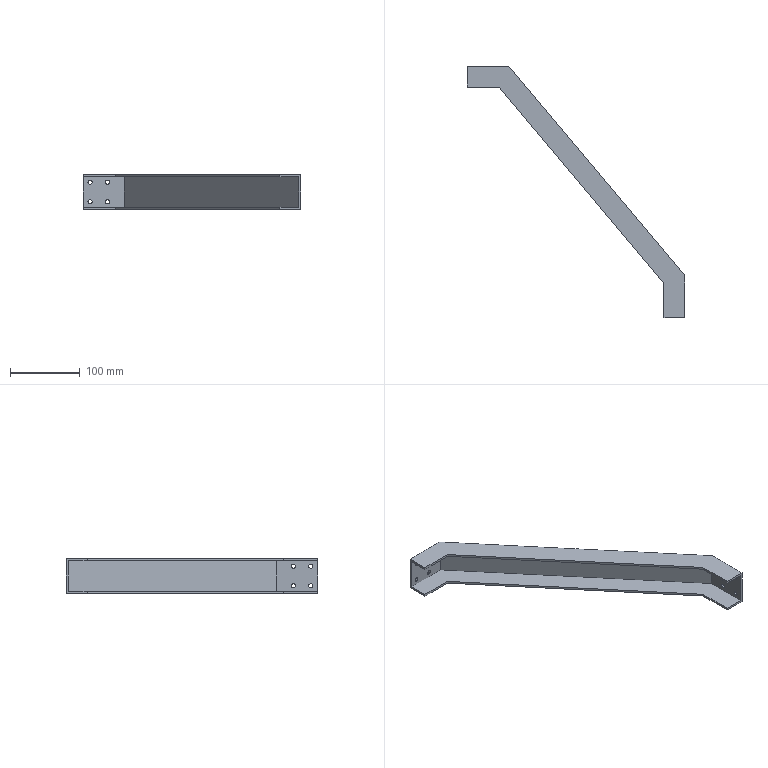Component | SolidWorks | BaffleFixingBracket-1 | 1 solid | 34 faces | box 311.73 x 360 x 50 mm | volume 154135 mm3 | plane 18 | cylinder 16 | commonest cylinder face diameters 6 x16
STEP:
#1=COLOUR_RGB('',0.7922,0.8196,0.9333);
#2=FILL_AREA_STYLE_COLOUR('',#1);
#3=FILL_AREA_STYLE('',(#2));
#4=SURFACE_STYLE_FILL_AREA(#3);
#5=SURFACE_SIDE_STYLE('',(#4));
#6=SURFACE_STYLE_USAGE(.BOTH.,#5);
#7=PRESENTATION_STYLE_ASSIGNMENT((#6));
#8=CARTESIAN_POINT('',(-24.578,20.455,-13.277));
#9=VERTEX_POINT('',#8);
#10=CARTESIAN_POINT('',(-24.342,20.455,-13.277));
#11=VERTEX_POINT('',#10);
#12=CARTESIAN_POINT('',(-24.46,20.455,-13.277));
#13=DIRECTION('',(0.,-1.,0.));
#14=DIRECTION('',(1.,0.,0.));
#15=AXIS2_PLACEMENT_3D('',#12,#13,#14);
#16=CIRCLE('',#15,0.1181);
#17=EDGE_CURVE('',#9,#11,#16,.T.);
#18=ORIENTED_EDGE('',*,*,#17,.F.);
#19=CARTESIAN_POINT('',(-24.578,20.337,-13.277));
#20=VERTEX_POINT('',#19);
#21=CARTESIAN_POINT('',(-24.578,20.455,-13.277));
#22=DIRECTION('',(0.,-1.,0.));
#23=VECTOR('',#22,39.37);
#24=LINE('',#21,#23);
#25=EDGE_CURVE('',#9,#20,#24,.T.);
#26=ORIENTED_EDGE('',*,*,#25,.T.);
#27=CARTESIAN_POINT('',(-24.342,20.337,-13.277));
#28=VERTEX_POINT('',#27);
#29=CARTESIAN_POINT('',(-24.46,20.337,-13.277));
#30=DIRECTION('',(0.,-1.,0.));
#31=DIRECTION('',(1.,0.,0.));
#32=AXIS2_PLACEMENT_3D('',#29,#30,#31);
#33=CIRCLE('',#32,0.1181);
#34=EDGE_CURVE('',#20,#28,#33,.T.);
#35=ORIENTED_EDGE('',*,*,#34,.T.);
#36=CARTESIAN_POINT('',(-24.342,20.455,-13.277));
#37=DIRECTION('',(0.,-1.,0.));
#38=VECTOR('',#37,39.37);
#39=LINE('',#36,#38);
#40=EDGE_CURVE('',#11,#28,#39,.T.);
#41=ORIENTED_EDGE('',*,*,#40,.F.);
#42=EDGE_LOOP('',(#18,#26,#35,#41));
#43=FACE_OUTER_BOUND('',#42,.T.);
#44=CARTESIAN_POINT('',(-24.46,20.455,-13.277));
#45=DIRECTION('',(0.,-1.,0.));
#46=DIRECTION('',(1.,0.,0.));
#47=AXIS2_PLACEMENT_3D('',#44,#45,#46);
#48=CYLINDRICAL_SURFACE('',#47,0.1181);
#49=ADVANCED_FACE('',(#43),#48,.F.);
#50=CARTESIAN_POINT('',(-24.578,20.455,-12.174));
#51=VERTEX_POINT('',#50);
#52=CARTESIAN_POINT('',(-24.342,20.455,-12.174));
#53=VERTEX_POINT('',#52);
#54=CARTESIAN_POINT('',(-24.46,20.455,-12.174));
#55=DIRECTION('',(0.,-1.,0.));
#56=DIRECTION('',(1.,0.,0.));
#57=AXIS2_PLACEMENT_3D('',#54,#55,#56);
#58=CIRCLE('',#57,0.1181);
#59=EDGE_CURVE('',#51,#53,#58,.T.);
#60=ORIENTED_EDGE('',*,*,#59,.F.);
#61=CARTESIAN_POINT('',(-24.578,20.337,-12.174));
#62=VERTEX_POINT('',#61);
#63=CARTESIAN_POINT('',(-24.578,20.455,-12.174));
#64=DIRECTION('',(0.,-1.,0.));
#65=VECTOR('',#64,39.37);
#66=LINE('',#63,#65);
#67=EDGE_CURVE('',#51,#62,#66,.T.);
#68=ORIENTED_EDGE('',*,*,#67,.T.);
#69=CARTESIAN_POINT('',(-24.342,20.337,-12.174));
#70=VERTEX_POINT('',#69);
#71=CARTESIAN_POINT('',(-24.46,20.337,-12.174));
#72=DIRECTION('',(0.,-1.,0.));
#73=DIRECTION('',(1.,0.,0.));
#74=AXIS2_PLACEMENT_3D('',#71,#72,#73);
#75=CIRCLE('',#74,0.1181);
#76=EDGE_CURVE('',#62,#70,#75,.T.);
#77=ORIENTED_EDGE('',*,*,#76,.T.);
#78=CARTESIAN_POINT('',(-24.342,20.455,-12.174));
#79=DIRECTION('',(0.,-1.,0.));
#80=VECTOR('',#79,39.37);
#81=LINE('',#78,#80);
#82=EDGE_CURVE('',#53,#70,#81,.T.);
#83=ORIENTED_EDGE('',*,*,#82,.F.);
#84=EDGE_LOOP('',(#60,#68,#77,#83));
#85=FACE_OUTER_BOUND('',#84,.T.);
#86=CARTESIAN_POINT('',(-24.46,20.455,-12.174));
#87=DIRECTION('',(0.,-1.,0.));
#88=DIRECTION('',(1.,0.,0.));
#89=AXIS2_PLACEMENT_3D('',#86,#87,#88);
#90=CYLINDRICAL_SURFACE('',#89,0.1181);
#91=ADVANCED_FACE('',(#85),#90,.F.);
#92=CARTESIAN_POINT('',(-23.594,20.455,-13.277));
#93=VERTEX_POINT('',#92);
#94=CARTESIAN_POINT('',(-23.357,20.455,-13.277));
#95=VERTEX_POINT('',#94);
#96=CARTESIAN_POINT('',(-23.476,20.455,-13.277));
#97=DIRECTION('',(0.,-1.,0.));
#98=DIRECTION('',(1.,0.,0.));
#99=AXIS2_PLACEMENT_3D('',#96,#97,#98);
#100=CIRCLE('',#99,0.1181);
#101=EDGE_CURVE('',#93,#95,#100,.T.);
#102=ORIENTED_EDGE('',*,*,#101,.F.);
#103=CARTESIAN_POINT('',(-23.594,20.337,-13.277));
#104=VERTEX_POINT('',#103);
#105=CARTESIAN_POINT('',(-23.594,20.455,-13.277));
#106=DIRECTION('',(0.,-1.,0.));
#107=VECTOR('',#106,39.37);
#108=LINE('',#105,#107);
#109=EDGE_CURVE('',#93,#104,#108,.T.);
#110=ORIENTED_EDGE('',*,*,#109,.T.);
#111=CARTESIAN_POINT('',(-23.357,20.337,-13.277));
#112=VERTEX_POINT('',#111);
#113=CARTESIAN_POINT('',(-23.476,20.337,-13.277));
#114=DIRECTION('',(0.,-1.,0.));
#115=DIRECTION('',(1.,0.,0.));
#116=AXIS2_PLACEMENT_3D('',#113,#114,#115);
#117=CIRCLE('',#116,0.1181);
#118=EDGE_CURVE('',#104,#112,#117,.T.);
#119=ORIENTED_EDGE('',*,*,#118,.T.);
#120=CARTESIAN_POINT('',(-23.357,20.455,-13.277));
#121=DIRECTION('',(0.,-1.,0.));
#122=VECTOR('',#121,39.37);
#123=LINE('',#120,#122);
#124=EDGE_CURVE('',#95,#112,#123,.T.);
#125=ORIENTED_EDGE('',*,*,#124,.F.);
#126=EDGE_LOOP('',(#102,#110,#119,#125));
#127=FACE_OUTER_BOUND('',#126,.T.);
#128=CARTESIAN_POINT('',(-23.476,20.455,-13.277));
#129=DIRECTION('',(0.,-1.,0.));
#130=DIRECTION('',(1.,0.,0.));
#131=AXIS2_PLACEMENT_3D('',#128,#129,#130);
#132=CYLINDRICAL_SURFACE('',#131,0.1181);
#133=ADVANCED_FACE('',(#127),#132,.F.);
#134=CARTESIAN_POINT('',(-23.594,20.455,-12.174));
#135=VERTEX_POINT('',#134);
#136=CARTESIAN_POINT('',(-23.357,20.455,-12.174));
#137=VERTEX_POINT('',#136);
#138=CARTESIAN_POINT('',(-23.476,20.455,-12.174));
#139=DIRECTION('',(0.,-1.,0.));
#140=DIRECTION('',(1.,0.,0.));
#141=AXIS2_PLACEMENT_3D('',#138,#139,#140);
#142=CIRCLE('',#141,0.1181);
#143=EDGE_CURVE('',#135,#137,#142,.T.);
#144=ORIENTED_EDGE('',*,*,#143,.F.);
#145=CARTESIAN_POINT('',(-23.594,20.337,-12.174));
#146=VERTEX_POINT('',#145);
#147=CARTESIAN_POINT('',(-23.594,20.455,-12.174));
#148=DIRECTION('',(0.,-1.,0.));
#149=VECTOR('',#148,39.37);
#150=LINE('',#147,#149);
#151=EDGE_CURVE('',#135,#146,#150,.T.);
#152=ORIENTED_EDGE('',*,*,#151,.T.);
#153=CARTESIAN_POINT('',(-23.357,20.337,-12.174));
#154=VERTEX_POINT('',#153);
#155=CARTESIAN_POINT('',(-23.476,20.337,-12.174));
#156=DIRECTION('',(0.,-1.,0.));
#157=DIRECTION('',(1.,0.,0.));
#158=AXIS2_PLACEMENT_3D('',#155,#156,#157);
#159=CIRCLE('',#158,0.1181);
#160=EDGE_CURVE('',#146,#154,#159,.T.);
#161=ORIENTED_EDGE('',*,*,#160,.T.);
#162=CARTESIAN_POINT('',(-23.357,20.455,-12.174));
#163=DIRECTION('',(0.,-1.,0.));
#164=VECTOR('',#163,39.37);
#165=LINE('',#162,#164);
#166=EDGE_CURVE('',#137,#154,#165,.T.);
#167=ORIENTED_EDGE('',*,*,#166,.F.);
#168=EDGE_LOOP('',(#144,#152,#161,#167));
#169=FACE_OUTER_BOUND('',#168,.T.);
#170=CARTESIAN_POINT('',(-23.476,20.455,-12.174));
#171=DIRECTION('',(0.,-1.,0.));
#172=DIRECTION('',(1.,0.,0.));
#173=AXIS2_PLACEMENT_3D('',#170,#171,#172);
#174=CYLINDRICAL_SURFACE('',#173,0.1181);
#175=ADVANCED_FACE('',(#169),#174,.F.);
#176=CARTESIAN_POINT('',(-12.581,6.794,-12.174));
#177=VERTEX_POINT('',#176);
#178=CARTESIAN_POINT('',(-12.581,6.558,-12.174));
#179=VERTEX_POINT('',#178);
#180=CARTESIAN_POINT('',(-12.581,6.676,-12.174));
#181=DIRECTION('',(-1.,0.,0.));
#182=DIRECTION('',(0.,-1.,0.));
#183=AXIS2_PLACEMENT_3D('',#180,#181,#182);
#184=CIRCLE('',#183,0.1181);
#185=EDGE_CURVE('',#177,#179,#184,.T.);
#186=ORIENTED_EDGE('',*,*,#185,.F.);
#187=CARTESIAN_POINT('',(-12.699,6.794,-12.174));
#188=VERTEX_POINT('',#187);
#189=CARTESIAN_POINT('',(-12.581,6.794,-12.174));
#190=DIRECTION('',(-1.,0.,0.));
#191=VECTOR('',#190,39.37);
#192=LINE('',#189,#191);
#193=EDGE_CURVE('',#177,#188,#192,.T.);
#194=ORIENTED_EDGE('',*,*,#193,.T.);
#195=CARTESIAN_POINT('',(-12.699,6.558,-12.174));
#196=VERTEX_POINT('',#195);
#197=CARTESIAN_POINT('',(-12.699,6.676,-12.174));
#198=DIRECTION('',(-1.,0.,0.));
#199=DIRECTION('',(0.,-1.,0.));
#200=AXIS2_PLACEMENT_3D('',#197,#198,#199);
#201=CIRCLE('',#200,0.1181);
#202=EDGE_CURVE('',#188,#196,#201,.T.);
#203=ORIENTED_EDGE('',*,*,#202,.T.);
#204=CARTESIAN_POINT('',(-12.581,6.558,-12.174));
#205=DIRECTION('',(-1.,0.,0.));
#206=VECTOR('',#205,39.37);
#207=LINE('',#204,#206);
#208=EDGE_CURVE('',#179,#196,#207,.T.);
#209=ORIENTED_EDGE('',*,*,#208,.F.);
#210=EDGE_LOOP('',(#186,#194,#203,#209));
#211=FACE_OUTER_BOUND('',#210,.T.);
#212=CARTESIAN_POINT('',(-12.581,6.676,-12.174));
#213=DIRECTION('',(-1.,0.,0.));
#214=DIRECTION('',(0.,-1.,0.));
#215=AXIS2_PLACEMENT_3D('',#212,#213,#214);
#216=CYLINDRICAL_SURFACE('',#215,0.1181);
#217=ADVANCED_FACE('',(#211),#216,.F.);
#218=CARTESIAN_POINT('',(-12.581,6.794,-13.277));
#219=VERTEX_POINT('',#218);
#220=CARTESIAN_POINT('',(-12.581,6.558,-13.277));
#221=VERTEX_POINT('',#220);
#222=CARTESIAN_POINT('',(-12.581,6.676,-13.277));
#223=DIRECTION('',(-1.,0.,0.));
#224=DIRECTION('',(0.,-1.,0.));
#225=AXIS2_PLACEMENT_3D('',#222,#223,#224);
#226=CIRCLE('',#225,0.1181);
#227=EDGE_CURVE('',#219,#221,#226,.T.);
#228=ORIENTED_EDGE('',*,*,#227,.F.);
#229=CARTESIAN_POINT('',(-12.699,6.794,-13.277));
#230=VERTEX_POINT('',#229);
#231=CARTESIAN_POINT('',(-12.581,6.794,-13.277));
#232=DIRECTION('',(-1.,0.,0.));
#233=VECTOR('',#232,39.37);
#234=LINE('',#231,#233);
#235=EDGE_CURVE('',#219,#230,#234,.T.);
#236=ORIENTED_EDGE('',*,*,#235,.T.);
#237=CARTESIAN_POINT('',(-12.699,6.558,-13.277));
#238=VERTEX_POINT('',#237);
#239=CARTESIAN_POINT('',(-12.699,6.676,-13.277));
#240=DIRECTION('',(-1.,0.,0.));
#241=DIRECTION('',(0.,-1.,0.));
#242=AXIS2_PLACEMENT_3D('',#239,#240,#241);
#243=CIRCLE('',#242,0.1181);
#244=EDGE_CURVE('',#230,#238,#243,.T.);
#245=ORIENTED_EDGE('',*,*,#244,.T.);
#246=CARTESIAN_POINT('',(-12.581,6.558,-13.277));
#247=DIRECTION('',(-1.,0.,0.));
#248=VECTOR('',#247,39.37);
#249=LINE('',#246,#248);
#250=EDGE_CURVE('',#221,#238,#249,.T.);
#251=ORIENTED_EDGE('',*,*,#250,.F.);
#252=EDGE_LOOP('',(#228,#236,#245,#251));
#253=FACE_OUTER_BOUND('',#252,.T.);
#254=CARTESIAN_POINT('',(-12.581,6.676,-13.277));
#255=DIRECTION('',(-1.,0.,0.));
#256=DIRECTION('',(0.,-1.,0.));
#257=AXIS2_PLACEMENT_3D('',#254,#255,#256);
#258=CYLINDRICAL_SURFACE('',#257,0.1181);
#259=ADVANCED_FACE('',(#253),#258,.F.);
#260=CARTESIAN_POINT('',(-12.581,7.778,-12.174));
#261=VERTEX_POINT('',#260);
#262=CARTESIAN_POINT('',(-12.581,7.542,-12.174));
#263=VERTEX_POINT('',#262);
#264=CARTESIAN_POINT('',(-12.581,7.66,-12.174));
#265=DIRECTION('',(-1.,0.,0.));
#266=DIRECTION('',(0.,-1.,0.));
#267=AXIS2_PLACEMENT_3D('',#264,#265,#266);
#268=CIRCLE('',#267,0.1181);
#269=EDGE_CURVE('',#261,#263,#268,.T.);
#270=ORIENTED_EDGE('',*,*,#269,.F.);
#271=CARTESIAN_POINT('',(-12.699,7.778,-12.174));
#272=VERTEX_POINT('',#271);
#273=CARTESIAN_POINT('',(-12.581,7.778,-12.174));
#274=DIRECTION('',(-1.,0.,0.));
#275=VECTOR('',#274,39.37);
#276=LINE('',#273,#275);
#277=EDGE_CURVE('',#261,#272,#276,.T.);
#278=ORIENTED_EDGE('',*,*,#277,.T.);
#279=CARTESIAN_POINT('',(-12.699,7.542,-12.174));
#280=VERTEX_POINT('',#279);
#281=CARTESIAN_POINT('',(-12.699,7.66,-12.174));
#282=DIRECTION('',(-1.,0.,0.));
#283=DIRECTION('',(0.,-1.,0.));
#284=AXIS2_PLACEMENT_3D('',#281,#282,#283);
#285=CIRCLE('',#284,0.1181);
#286=EDGE_CURVE('',#272,#280,#285,.T.);
#287=ORIENTED_EDGE('',*,*,#286,.T.);
#288=CARTESIAN_POINT('',(-12.581,7.542,-12.174));
#289=DIRECTION('',(-1.,0.,0.));
#290=VECTOR('',#289,39.37);
#291=LINE('',#288,#290);
#292=EDGE_CURVE('',#263,#280,#291,.T.);
#293=ORIENTED_EDGE('',*,*,#292,.F.);
#294=EDGE_LOOP('',(#270,#278,#287,#293));
#295=FACE_OUTER_BOUND('',#294,.T.);
#296=CARTESIAN_POINT('',(-12.581,7.66,-12.174));
#297=DIRECTION('',(-1.,0.,0.));
#298=DIRECTION('',(0.,-1.,0.));
#299=AXIS2_PLACEMENT_3D('',#296,#297,#298);
#300=CYLINDRICAL_SURFACE('',#299,0.1181);
#301=ADVANCED_FACE('',(#295),#300,.F.);
#302=CARTESIAN_POINT('',(-12.581,7.778,-13.277));
#303=VERTEX_POINT('',#302);
#304=CARTESIAN_POINT('',(-12.581,7.542,-13.277));
#305=VERTEX_POINT('',#304);
#306=CARTESIAN_POINT('',(-12.581,7.66,-13.277));
#307=DIRECTION('',(-1.,0.,0.));
#308=DIRECTION('',(0.,-1.,0.));
#309=AXIS2_PLACEMENT_3D('',#306,#307,#308);
#310=CIRCLE('',#309,0.1181);
#311=EDGE_CURVE('',#303,#305,#310,.T.);
#312=ORIENTED_EDGE('',*,*,#311,.F.);
#313=CARTESIAN_POINT('',(-12.699,7.778,-13.277));
#314=VERTEX_POINT('',#313);
#315=CARTESIAN_POINT('',(-12.581,7.778,-13.277));
#316=DIRECTION('',(-1.,0.,0.));
#317=VECTOR('',#316,39.37);
#318=LINE('',#315,#317);
#319=EDGE_CURVE('',#303,#314,#318,.T.);
#320=ORIENTED_EDGE('',*,*,#319,.T.);
#321=CARTESIAN_POINT('',(-12.699,7.542,-13.277));
#322=VERTEX_POINT('',#321);
#323=CARTESIAN_POINT('',(-12.699,7.66,-13.277));
#324=DIRECTION('',(-1.,0.,0.));
#325=DIRECTION('',(0.,-1.,0.));
#326=AXIS2_PLACEMENT_3D('',#323,#324,#325);
#327=CIRCLE('',#326,0.1181);
#328=EDGE_CURVE('',#314,#322,#327,.T.);
#329=ORIENTED_EDGE('',*,*,#328,.T.);
#330=CARTESIAN_POINT('',(-12.581,7.542,-13.277));
#331=DIRECTION('',(-1.,0.,0.));
#332=VECTOR('',#331,39.37);
#333=LINE('',#330,#332);
#334=EDGE_CURVE('',#305,#322,#333,.T.);
#335=ORIENTED_EDGE('',*,*,#334,.F.);
#336=EDGE_LOOP('',(#312,#320,#329,#335));
#337=FACE_OUTER_BOUND('',#336,.T.);
#338=CARTESIAN_POINT('',(-12.581,7.66,-13.277));
#339=DIRECTION('',(-1.,0.,0.));
#340=DIRECTION('',(0.,-1.,0.));
#341=AXIS2_PLACEMENT_3D('',#338,#339,#340);
#342=CYLINDRICAL_SURFACE('',#341,0.1181);
#343=ADVANCED_FACE('',(#337),#342,.F.);
#344=CARTESIAN_POINT('',(-24.854,19.274,-13.592));
#345=VERTEX_POINT('',#344);
#346=CARTESIAN_POINT('',(-24.854,19.274,-13.71));
#347=VERTEX_POINT('',#346);
#348=CARTESIAN_POINT('',(-24.854,19.274,-11.741));
#349=DIRECTION('',(0.,0.,-1.));
#350=VECTOR('',#349,39.37);
#351=LINE('',#348,#350);
#352=EDGE_CURVE('',#345,#347,#351,.T.);
#353=ORIENTED_EDGE('',*,*,#352,.F.);
#354=CARTESIAN_POINT('',(-24.854,20.337,-13.592));
#355=VERTEX_POINT('',#354);
#356=CARTESIAN_POINT('',(-24.854,18.273,-13.592));
#357=DIRECTION('',(0.,1.,0.));
#358=VECTOR('',#357,39.37);
#359=LINE('',#356,#358);
#360=EDGE_CURVE('',#345,#355,#359,.T.);
#361=ORIENTED_EDGE('',*,*,#360,.T.);
#362=CARTESIAN_POINT('',(-24.854,20.337,-11.859));
#363=VERTEX_POINT('',#362);
#364=CARTESIAN_POINT('',(-24.854,20.337,-11.741));
#365=DIRECTION('',(0.,0.,-1.));
#366=VECTOR('',#365,39.37);
#367=LINE('',#364,#366);
#368=EDGE_CURVE('',#363,#355,#367,.T.);
#369=ORIENTED_EDGE('',*,*,#368,.F.);
#370=CARTESIAN_POINT('',(-24.854,19.274,-11.859));
#371=VERTEX_POINT('',#370);
#372=CARTESIAN_POINT('',(-24.854,18.273,-11.859));
#373=DIRECTION('',(0.,1.,0.));
#374=VECTOR('',#373,39.37);
#375=LINE('',#372,#374);
#376=EDGE_CURVE('',#371,#363,#375,.T.);
#377=ORIENTED_EDGE('',*,*,#376,.F.);
#378=CARTESIAN_POINT('',(-24.854,19.274,-11.741));
#379=VERTEX_POINT('',#378);
#380=CARTESIAN_POINT('',(-24.854,19.274,-11.741));
#381=DIRECTION('',(0.,0.,-1.));
#382=VECTOR('',#381,39.37);
#383=LINE('',#380,#382);
#384=EDGE_CURVE('',#379,#371,#383,.T.);
#385=ORIENTED_EDGE('',*,*,#384,.F.);
#386=CARTESIAN_POINT('',(-24.854,20.455,-11.741));
#387=VERTEX_POINT('',#386);
#388=CARTESIAN_POINT('',(-24.854,19.274,-11.741));
#389=DIRECTION('',(0.,1.,0.));
#390=VECTOR('',#389,39.37);
#391=LINE('',#388,#390);
#392=EDGE_CURVE('',#379,#387,#391,.T.);
#393=ORIENTED_EDGE('',*,*,#392,.T.);
#394=CARTESIAN_POINT('',(-24.854,20.455,-13.71));
#395=VERTEX_POINT('',#394);
#396=CARTESIAN_POINT('',(-24.854,20.455,-11.741));
#397=DIRECTION('',(0.,0.,-1.));
#398=VECTOR('',#397,39.37);
#399=LINE('',#396,#398);
#400=EDGE_CURVE('',#387,#395,#399,.T.);
#401=ORIENTED_EDGE('',*,*,#400,.T.);
#402=CARTESIAN_POINT('',(-24.854,19.274,-13.71));
#403=DIRECTION('',(0.,1.,0.));
#404=VECTOR('',#403,39.37);
#405=LINE('',#402,#404);
#406=EDGE_CURVE('',#347,#395,#405,.T.);
#407=ORIENTED_EDGE('',*,*,#406,.F.);
#408=EDGE_LOOP('',(#353,#361,#369,#377,#385,#393,#401,#407));
#409=FACE_OUTER_BOUND('',#408,.T.);
#410=CARTESIAN_POINT('',(-24.854,19.274,-11.741));
#411=DIRECTION('',(-1.,0.,0.));
#412=DIRECTION('',(0.,0.,1.));
#413=AXIS2_PLACEMENT_3D('',#410,#411,#412);
#414=PLANE('',#413);
#415=ADVANCED_FACE('',(#409),#414,.T.);
#416=CARTESIAN_POINT('',(-23.042,19.274,-13.592));
#417=VERTEX_POINT('',#416);
#418=CARTESIAN_POINT('',(-23.042,19.274,-13.71));
#419=VERTEX_POINT('',#418);
#420=CARTESIAN_POINT('',(-23.042,19.274,-11.741));
#421=DIRECTION('',(0.,0.,-1.));
#422=VECTOR('',#421,39.37);
#423=LINE('',#420,#422);
#424=EDGE_CURVE('',#417,#419,#423,.T.);
#425=ORIENTED_EDGE('',*,*,#424,.F.);
#426=CARTESIAN_POINT('',(-17.321,19.274,-13.592));
#427=DIRECTION('',(-1.,-0.,0.));
#428=VECTOR('',#427,39.37);
#429=LINE('',#426,#428);
#430=EDGE_CURVE('',#417,#345,#429,.T.);
#431=ORIENTED_EDGE('',*,*,#430,.T.);
#432=ORIENTED_EDGE('',*,*,#352,.T.);
#433=CARTESIAN_POINT('',(-22.491,19.274,-13.71));
#434=DIRECTION('',(-1.,-0.,0.));
#435=VECTOR('',#434,39.37);
#436=LINE('',#433,#435);
#437=EDGE_CURVE('',#419,#347,#436,.T.);
#438=ORIENTED_EDGE('',*,*,#437,.F.);
#439=EDGE_LOOP('',(#425,#431,#432,#438));
#440=FACE_OUTER_BOUND('',#439,.T.);
#441=CARTESIAN_POINT('',(-22.491,19.274,-11.741));
#442=DIRECTION('',(0.,-1.,0.));
#443=DIRECTION('',(1.,0.,0.));
#444=AXIS2_PLACEMENT_3D('',#441,#442,#443);
#445=PLANE('',#444);
#446=ADVANCED_FACE('',(#440),#445,.T.);
#447=CARTESIAN_POINT('',(-13.762,8.214,-13.592));
#448=VERTEX_POINT('',#447);
#449=CARTESIAN_POINT('',(-13.762,8.214,-13.71));
#450=VERTEX_POINT('',#449);
#451=CARTESIAN_POINT('',(-13.762,8.214,-11.741));
#452=DIRECTION('',(0.,0.,-1.));
#453=VECTOR('',#452,39.37);
#454=LINE('',#451,#453);
#455=EDGE_CURVE('',#448,#450,#454,.T.);
#456=ORIENTED_EDGE('',*,*,#455,.F.);
#457=CARTESIAN_POINT('',(-20.185,15.87,-13.592));
#458=DIRECTION('',(-0.6428,0.766,0.));
#459=VECTOR('',#458,39.37);
#460=LINE('',#457,#459);
#461=EDGE_CURVE('',#448,#417,#460,.T.);
#462=ORIENTED_EDGE('',*,*,#461,.T.);
#463=ORIENTED_EDGE('',*,*,#424,.T.);
#464=CARTESIAN_POINT('',(-13.485,7.885,-13.71));
#465=DIRECTION('',(-0.6428,0.766,0.));
#466=VECTOR('',#465,39.37);
#467=LINE('',#464,#466);
#468=EDGE_CURVE('',#450,#419,#467,.T.);
#469=ORIENTED_EDGE('',*,*,#468,.F.);
#470=EDGE_LOOP('',(#456,#462,#463,#469));
#471=FACE_OUTER_BOUND('',#470,.T.);
#472=CARTESIAN_POINT('',(-13.485,7.885,-11.741));
#473=DIRECTION('',(-0.766,-0.6428,0.));
#474=DIRECTION('',(0.6428,-0.766,0.));
#475=AXIS2_PLACEMENT_3D('',#472,#473,#474);
#476=PLANE('',#475);
#477=ADVANCED_FACE('',(#471),#476,.T.);
#478=CARTESIAN_POINT('',(-13.762,6.282,-13.592));
#479=VERTEX_POINT('',#478);
#480=CARTESIAN_POINT('',(-13.762,6.282,-13.71));
#481=VERTEX_POINT('',#480);
#482=CARTESIAN_POINT('',(-13.762,6.282,-11.741));
#483=DIRECTION('',(0.,0.,-1.));
#484=VECTOR('',#483,39.37);
#485=LINE('',#482,#484);
#486=EDGE_CURVE('',#479,#481,#485,.T.);
#487=ORIENTED_EDGE('',*,*,#486,.F.);
#488=CARTESIAN_POINT('',(-13.762,18.273,-13.592));
#489=DIRECTION('',(0.,1.,0.));
#490=VECTOR('',#489,39.37);
#491=LINE('',#488,#490);
#492=EDGE_CURVE('',#479,#448,#491,.T.);
#493=ORIENTED_EDGE('',*,*,#492,.T.);
#494=ORIENTED_EDGE('',*,*,#455,.T.);
#495=CARTESIAN_POINT('',(-13.762,6.282,-13.71));
#496=DIRECTION('',(0.,1.,0.));
#497=VECTOR('',#496,39.37);
#498=LINE('',#495,#497);
#499=EDGE_CURVE('',#481,#450,#498,.T.);
#500=ORIENTED_EDGE('',*,*,#499,.F.);
#501=EDGE_LOOP('',(#487,#493,#494,#500));
#502=FACE_OUTER_BOUND('',#501,.T.);
#503=CARTESIAN_POINT('',(-13.762,6.282,-11.741));
#504=DIRECTION('',(-1.,0.,0.));
#505=DIRECTION('',(-0.,-1.,0.));
#506=AXIS2_PLACEMENT_3D('',#503,#504,#505);
#507=PLANE('',#506);
#508=ADVANCED_FACE('',(#502),#507,.T.);
#509=CARTESIAN_POINT('',(-12.699,6.282,-11.859));
#510=VERTEX_POINT('',#509);
#511=CARTESIAN_POINT('',(-12.699,6.282,-13.592));
#512=VERTEX_POINT('',#511);
#513=CARTESIAN_POINT('',(-12.699,6.282,-11.741));
#514=DIRECTION('',(0.,0.,-1.));
#515=VECTOR('',#514,39.37);
#516=LINE('',#513,#515);
#517=EDGE_CURVE('',#510,#512,#516,.T.);
#518=ORIENTED_EDGE('',*,*,#517,.T.);
#519=CARTESIAN_POINT('',(-17.321,6.282,-13.592));
#520=DIRECTION('',(-1.,0.,0.));
#521=VECTOR('',#520,39.37);
#522=LINE('',#519,#521);
#523=EDGE_CURVE('',#512,#479,#522,.T.);
#524=ORIENTED_EDGE('',*,*,#523,.T.);
#525=ORIENTED_EDGE('',*,*,#486,.T.);
#526=CARTESIAN_POINT('',(-12.581,6.282,-13.71));
#527=VERTEX_POINT('',#526);
#528=CARTESIAN_POINT('',(-12.581,6.282,-13.71));
#529=DIRECTION('',(-1.,0.,0.));
#530=VECTOR('',#529,39.37);
#531=LINE('',#528,#530);
#532=EDGE_CURVE('',#527,#481,#531,.T.);
#533=ORIENTED_EDGE('',*,*,#532,.F.);
#534=CARTESIAN_POINT('',(-12.581,6.282,-11.741));
#535=VERTEX_POINT('',#534);
#536=CARTESIAN_POINT('',(-12.581,6.282,-11.741));
#537=DIRECTION('',(0.,0.,-1.));
#538=VECTOR('',#537,39.37);
#539=LINE('',#536,#538);
#540=EDGE_CURVE('',#535,#527,#539,.T.);
#541=ORIENTED_EDGE('',*,*,#540,.F.);
#542=CARTESIAN_POINT('',(-13.762,6.282,-11.741));
#543=VERTEX_POINT('',#542);
#544=CARTESIAN_POINT('',(-12.581,6.282,-11.741));
#545=DIRECTION('',(-1.,0.,0.));
#546=VECTOR('',#545,39.37);
#547=LINE('',#544,#546);
#548=EDGE_CURVE('',#535,#543,#547,.T.);
#549=ORIENTED_EDGE('',*,*,#548,.T.);
#550=CARTESIAN_POINT('',(-13.762,6.282,-11.859));
#551=VERTEX_POINT('',#550);
#552=CARTESIAN_POINT('',(-13.762,6.282,-11.741));
#553=DIRECTION('',(0.,0.,-1.));
#554=VECTOR('',#553,39.37);
#555=LINE('',#552,#554);
#556=EDGE_CURVE('',#543,#551,#555,.T.);
#557=ORIENTED_EDGE('',*,*,#556,.T.);
#558=CARTESIAN_POINT('',(-17.321,6.282,-11.859));
#559=DIRECTION('',(-1.,0.,0.));
#560=VECTOR('',#559,39.37);
#561=LINE('',#558,#560);
#562=EDGE_CURVE('',#510,#551,#561,.T.);
#563=ORIENTED_EDGE('',*,*,#562,.F.);
#564=EDGE_LOOP('',(#518,#524,#525,#533,#541,#549,#557,#563));
#565=FACE_OUTER_BOUND('',#564,.T.);
#566=CARTESIAN_POINT('',(-12.581,6.282,-11.741));
#567=DIRECTION('',(0.,-1.,0.));
#568=DIRECTION('',(0.,0.,-1.));
#569=AXIS2_PLACEMENT_3D('',#566,#567,#568);
#570=PLANE('',#569);
#571=ADVANCED_FACE('',(#565),#570,.T.);
#572=CARTESIAN_POINT('',(-24.46,20.455,-13.277));
#573=DIRECTION('',(0.,-1.,0.));
#574=DIRECTION('',(1.,0.,0.));
#575=AXIS2_PLACEMENT_3D('',#572,#573,#574);
#576=CIRCLE('',#575,0.1181);
#577=EDGE_CURVE('',#11,#9,#576,.T.);
#578=ORIENTED_EDGE('',*,*,#577,.T.);
#579=ORIENTED_EDGE('',*,*,#17,.T.);
#580=EDGE_LOOP('',(#578,#579));
#581=FACE_BOUND('',#580,.T.);
#582=CARTESIAN_POINT('',(-24.46,20.455,-12.174));
#583=DIRECTION('',(0.,-1.,0.));
#584=DIRECTION('',(1.,0.,0.));
#585=AXIS2_PLACEMENT_3D('',#582,#583,#584);
#586=CIRCLE('',#585,0.1181);
#587=EDGE_CURVE('',#53,#51,#586,.T.);
#588=ORIENTED_EDGE('',*,*,#587,.T.);
#589=ORIENTED_EDGE('',*,*,#59,.T.);
#590=EDGE_LOOP('',(#588,#589));
#591=FACE_BOUND('',#590,.T.);
#592=CARTESIAN_POINT('',(-23.476,20.455,-13.277));
#593=DIRECTION('',(0.,-1.,0.));
#594=DIRECTION('',(1.,0.,0.));
#595=AXIS2_PLACEMENT_3D('',#592,#593,#594);
#596=CIRCLE('',#595,0.1181);
#597=EDGE_CURVE('',#95,#93,#596,.T.);
#598=ORIENTED_EDGE('',*,*,#597,.T.);
#599=ORIENTED_EDGE('',*,*,#101,.T.);
#600=EDGE_LOOP('',(#598,#599));
#601=FACE_BOUND('',#600,.T.);
#602=CARTESIAN_POINT('',(-23.476,20.455,-12.174));
#603=DIRECTION('',(0.,-1.,0.));
#604=DIRECTION('',(1.,0.,0.));
#605=AXIS2_PLACEMENT_3D('',#602,#603,#604);
#606=CIRCLE('',#605,0.1181);
#607=EDGE_CURVE('',#137,#135,#606,.T.);
#608=ORIENTED_EDGE('',*,*,#607,.T.);
#609=ORIENTED_EDGE('',*,*,#143,.T.);
#610=EDGE_LOOP('',(#608,#609));
#611=FACE_BOUND('',#610,.T.);
#612=CARTESIAN_POINT('',(-22.491,20.455,-13.71));
#613=VERTEX_POINT('',#612);
#614=CARTESIAN_POINT('',(-22.491,20.455,-13.71));
#615=DIRECTION('',(-1.,-0.,0.));
#616=VECTOR('',#615,39.37);
#617=LINE('',#614,#616);
#618=EDGE_CURVE('',#613,#395,#617,.T.);
#619=ORIENTED_EDGE('',*,*,#618,.T.);
#620=ORIENTED_EDGE('',*,*,#400,.F.);
#621=CARTESIAN_POINT('',(-22.491,20.455,-11.741));
#622=VERTEX_POINT('',#621);
#623=CARTESIAN_POINT('',(-22.491,20.455,-11.741));
#624=DIRECTION('',(-1.,-0.,0.));
#625=VECTOR('',#624,39.37);
#626=LINE('',#623,#625);
#627=EDGE_CURVE('',#622,#387,#626,.T.);
#628=ORIENTED_EDGE('',*,*,#627,.F.);
#629=CARTESIAN_POINT('',(-22.491,20.455,-11.741));
#630=DIRECTION('',(0.,0.,-1.));
#631=VECTOR('',#630,39.37);
#632=LINE('',#629,#631);
#633=EDGE_CURVE('',#622,#613,#632,.T.);
#634=ORIENTED_EDGE('',*,*,#633,.T.);
#635=EDGE_LOOP('',(#619,#620,#628,#634));
#636=FACE_OUTER_BOUND('',#635,.T.);
#637=CARTESIAN_POINT('',(-22.491,20.455,-11.741));
#638=DIRECTION('',(0.,-1.,0.));
#639=DIRECTION('',(1.,0.,0.));
#640=AXIS2_PLACEMENT_3D('',#637,#638,#639);
#641=PLANE('',#640);
#642=ADVANCED_FACE('',(#581,#591,#601,#611,#636),#641,.F.);
#643=CARTESIAN_POINT('',(-23.042,19.274,-11.859));
#644=VERTEX_POINT('',#643);
#645=CARTESIAN_POINT('',(-17.321,19.274,-11.859));
#646=DIRECTION('',(-1.,-0.,0.));
#647=VECTOR('',#646,39.37);
#648=LINE('',#645,#647);
#649=EDGE_CURVE('',#644,#371,#648,.T.);
#650=ORIENTED_EDGE('',*,*,#649,.F.);
#651=CARTESIAN_POINT('',(-23.042,19.274,-11.741));
#652=VERTEX_POINT('',#651);
#653=CARTESIAN_POINT('',(-23.042,19.274,-11.741));
#654=DIRECTION('',(0.,0.,-1.));
#655=VECTOR('',#654,39.37);
#656=LINE('',#653,#655);
#657=EDGE_CURVE('',#652,#644,#656,.T.);
#658=ORIENTED_EDGE('',*,*,#657,.F.);
#659=CARTESIAN_POINT('',(-22.491,19.274,-11.741));
#660=DIRECTION('',(-1.,-0.,0.));
#661=VECTOR('',#660,39.37);
#662=LINE('',#659,#661);
#663=EDGE_CURVE('',#652,#379,#662,.T.);
#664=ORIENTED_EDGE('',*,*,#663,.T.);
#665=ORIENTED_EDGE('',*,*,#384,.T.);
#666=EDGE_LOOP('',(#650,#658,#664,#665));
#667=FACE_OUTER_BOUND('',#666,.T.);
#668=CARTESIAN_POINT('',(-22.491,19.274,-11.741));
#669=DIRECTION('',(0.,-1.,0.));
#670=DIRECTION('',(1.,0.,0.));
#671=AXIS2_PLACEMENT_3D('',#668,#669,#670);
#672=PLANE('',#671);
#673=ADVANCED_FACE('',(#667),#672,.T.);
#674=CARTESIAN_POINT('',(-13.762,8.214,-11.859));
#675=VERTEX_POINT('',#674);
#676=CARTESIAN_POINT('',(-20.185,15.87,-11.859));
#677=DIRECTION('',(-0.6428,0.766,0.));
#678=VECTOR('',#677,39.37);
#679=LINE('',#676,#678);
#680=EDGE_CURVE('',#675,#644,#679,.T.);
#681=ORIENTED_EDGE('',*,*,#680,.F.);
#682=CARTESIAN_POINT('',(-13.762,8.214,-11.741));
#683=VERTEX_POINT('',#682);
#684=CARTESIAN_POINT('',(-13.762,8.214,-11.741));
#685=DIRECTION('',(0.,0.,-1.));
#686=VECTOR('',#685,39.37);
#687=LINE('',#684,#686);
#688=EDGE_CURVE('',#683,#675,#687,.T.);
#689=ORIENTED_EDGE('',*,*,#688,.F.);
#690=CARTESIAN_POINT('',(-13.485,7.885,-11.741));
#691=DIRECTION('',(-0.6428,0.766,0.));
#692=VECTOR('',#691,39.37);
#693=LINE('',#690,#692);
#694=EDGE_CURVE('',#683,#652,#693,.T.);
#695=ORIENTED_EDGE('',*,*,#694,.T.);
#696=ORIENTED_EDGE('',*,*,#657,.T.);
#697=EDGE_LOOP('',(#681,#689,#695,#696));
#698=FACE_OUTER_BOUND('',#697,.T.);
#699=CARTESIAN_POINT('',(-13.485,7.885,-11.741));
#700=DIRECTION('',(-0.766,-0.6428,0.));
#701=DIRECTION('',(0.6428,-0.766,0.));
#702=AXIS2_PLACEMENT_3D('',#699,#700,#701);
#703=PLANE('',#702);
#704=ADVANCED_FACE('',(#698),#703,.T.);
#705=CARTESIAN_POINT('',(-13.762,18.273,-11.859));
#706=DIRECTION('',(0.,1.,0.));
#707=VECTOR('',#706,39.37);
#708=LINE('',#705,#707);
#709=EDGE_CURVE('',#551,#675,#708,.T.);
#710=ORIENTED_EDGE('',*,*,#709,.F.);
#711=ORIENTED_EDGE('',*,*,#556,.F.);
#712=CARTESIAN_POINT('',(-13.762,6.282,-11.741));
#713=DIRECTION('',(0.,1.,0.));
#714=VECTOR('',#713,39.37);
#715=LINE('',#712,#714);
#716=EDGE_CURVE('',#543,#683,#715,.T.);
#717=ORIENTED_EDGE('',*,*,#716,.T.);
#718=ORIENTED_EDGE('',*,*,#688,.T.);
#719=EDGE_LOOP('',(#710,#711,#717,#718));
#720=FACE_OUTER_BOUND('',#719,.T.);
#721=CARTESIAN_POINT('',(-13.762,6.282,-11.741));
#722=DIRECTION('',(-1.,0.,0.));
#723=DIRECTION('',(-0.,-1.,0.));
#724=AXIS2_PLACEMENT_3D('',#721,#722,#723);
#725=PLANE('',#724);
#726=ADVANCED_FACE('',(#720),#725,.T.);
#727=CARTESIAN_POINT('',(-12.581,6.676,-12.174));
#728=DIRECTION('',(-1.,0.,0.));
#729=DIRECTION('',(0.,-1.,0.));
#730=AXIS2_PLACEMENT_3D('',#727,#728,#729);
#731=CIRCLE('',#730,0.1181);
#732=EDGE_CURVE('',#179,#177,#731,.T.);
#733=ORIENTED_EDGE('',*,*,#732,.T.);
#734=ORIENTED_EDGE('',*,*,#185,.T.);
#735=EDGE_LOOP('',(#733,#734));
#736=FACE_BOUND('',#735,.T.);
#737=CARTESIAN_POINT('',(-12.581,6.676,-13.277));
#738=DIRECTION('',(-1.,0.,0.));
#739=DIRECTION('',(0.,-1.,0.));
#740=AXIS2_PLACEMENT_3D('',#737,#738,#739);
#741=CIRCLE('',#740,0.1181);
#742=EDGE_CURVE('',#221,#219,#741,.T.);
#743=ORIENTED_EDGE('',*,*,#742,.T.);
#744=ORIENTED_EDGE('',*,*,#227,.T.);
#745=EDGE_LOOP('',(#743,#744));
#746=FACE_BOUND('',#745,.T.);
#747=CARTESIAN_POINT('',(-12.581,7.66,-12.174));
#748=DIRECTION('',(-1.,0.,0.));
#749=DIRECTION('',(0.,-1.,0.));
#750=AXIS2_PLACEMENT_3D('',#747,#748,#749);
#751=CIRCLE('',#750,0.1181);
#752=EDGE_CURVE('',#263,#261,#751,.T.);
#753=ORIENTED_EDGE('',*,*,#752,.T.);
#754=ORIENTED_EDGE('',*,*,#269,.T.);
#755=EDGE_LOOP('',(#753,#754));
#756=FACE_BOUND('',#755,.T.);
#757=CARTESIAN_POINT('',(-12.581,7.66,-13.277));
#758=DIRECTION('',(-1.,0.,0.));
#759=DIRECTION('',(0.,-1.,0.));
#760=AXIS2_PLACEMENT_3D('',#757,#758,#759);
#761=CIRCLE('',#760,0.1181);
#762=EDGE_CURVE('',#305,#303,#761,.T.);
#763=ORIENTED_EDGE('',*,*,#762,.T.);
#764=ORIENTED_EDGE('',*,*,#311,.T.);
#765=EDGE_LOOP('',(#763,#764));
#766=FACE_BOUND('',#765,.T.);
#767=CARTESIAN_POINT('',(-12.581,8.644,-13.71));
#768=VERTEX_POINT('',#767);
#769=CARTESIAN_POINT('',(-12.581,6.282,-13.71));
#770=DIRECTION('',(0.,1.,0.));
#771=VECTOR('',#770,39.37);
#772=LINE('',#769,#771);
#773=EDGE_CURVE('',#527,#768,#772,.T.);
#774=ORIENTED_EDGE('',*,*,#773,.T.);
#775=CARTESIAN_POINT('',(-12.581,8.644,-11.741));
#776=VERTEX_POINT('',#775);
#777=CARTESIAN_POINT('',(-12.581,8.644,-11.741));
#778=DIRECTION('',(0.,0.,-1.));
#779=VECTOR('',#778,39.37);
#780=LINE('',#777,#779);
#781=EDGE_CURVE('',#776,#768,#780,.T.);
#782=ORIENTED_EDGE('',*,*,#781,.F.);
#783=CARTESIAN_POINT('',(-12.581,6.282,-11.741));
#784=DIRECTION('',(0.,1.,0.));
#785=VECTOR('',#784,39.37);
#786=LINE('',#783,#785);
#787=EDGE_CURVE('',#535,#776,#786,.T.);
#788=ORIENTED_EDGE('',*,*,#787,.F.);
#789=ORIENTED_EDGE('',*,*,#540,.T.);
#790=EDGE_LOOP('',(#774,#782,#788,#789));
#791=FACE_OUTER_BOUND('',#790,.T.);
#792=CARTESIAN_POINT('',(-12.581,6.282,-11.741));
#793=DIRECTION('',(-1.,0.,0.));
#794=DIRECTION('',(-0.,-1.,0.));
#795=AXIS2_PLACEMENT_3D('',#792,#793,#794);
#796=PLANE('',#795);
#797=ADVANCED_FACE('',(#736,#746,#756,#766,#791),#796,.F.);
#798=CARTESIAN_POINT('',(-12.581,8.644,-13.71));
#799=DIRECTION('',(-0.6428,0.766,0.));
#800=VECTOR('',#799,39.37);
#801=LINE('',#798,#800);
#802=EDGE_CURVE('',#768,#613,#801,.T.);
#803=ORIENTED_EDGE('',*,*,#802,.T.);
#804=ORIENTED_EDGE('',*,*,#633,.F.);
#805=CARTESIAN_POINT('',(-12.581,8.644,-11.741));
#806=DIRECTION('',(-0.6428,0.766,0.));
#807=VECTOR('',#806,39.37);
#808=LINE('',#805,#807);
#809=EDGE_CURVE('',#776,#622,#808,.T.);
#810=ORIENTED_EDGE('',*,*,#809,.F.);
#811=ORIENTED_EDGE('',*,*,#781,.T.);
#812=EDGE_LOOP('',(#803,#804,#810,#811));
#813=FACE_OUTER_BOUND('',#812,.T.);
#814=CARTESIAN_POINT('',(-12.581,8.644,-11.741));
#815=DIRECTION('',(-0.766,-0.6428,0.));
#816=DIRECTION('',(0.6428,-0.766,0.));
#817=AXIS2_PLACEMENT_3D('',#814,#815,#816);
#818=PLANE('',#817);
#819=ADVANCED_FACE('',(#813),#818,.F.);
#820=ORIENTED_EDGE('',*,*,#627,.T.);
#821=ORIENTED_EDGE('',*,*,#392,.F.);
#822=ORIENTED_EDGE('',*,*,#663,.F.);
#823=ORIENTED_EDGE('',*,*,#694,.F.);
#824=ORIENTED_EDGE('',*,*,#716,.F.);
#825=ORIENTED_EDGE('',*,*,#548,.F.);
#826=ORIENTED_EDGE('',*,*,#787,.T.);
#827=ORIENTED_EDGE('',*,*,#809,.T.);
#828=EDGE_LOOP('',(#820,#821,#822,#823,#824,#825,#826,#827));
#829=FACE_OUTER_BOUND('',#828,.T.);
#830=CARTESIAN_POINT('',(-17.321,18.273,-11.741));
#831=DIRECTION('',(0.,0.,-1.));
#832=DIRECTION('',(-1.,0.,0.));
#833=AXIS2_PLACEMENT_3D('',#830,#831,#832);
#834=PLANE('',#833);
#835=ADVANCED_FACE('',(#829),#834,.F.);
#836=ORIENTED_EDGE('',*,*,#618,.F.);
#837=ORIENTED_EDGE('',*,*,#802,.F.);
#838=ORIENTED_EDGE('',*,*,#773,.F.);
#839=ORIENTED_EDGE('',*,*,#532,.T.);
#840=ORIENTED_EDGE('',*,*,#499,.T.);
#841=ORIENTED_EDGE('',*,*,#468,.T.);
#842=ORIENTED_EDGE('',*,*,#437,.T.);
#843=ORIENTED_EDGE('',*,*,#406,.T.);
#844=EDGE_LOOP('',(#836,#837,#838,#839,#840,#841,#842,#843));
#845=FACE_OUTER_BOUND('',#844,.T.);
#846=CARTESIAN_POINT('',(-17.321,18.273,-13.71));
#847=DIRECTION('',(0.,0.,-1.));
#848=DIRECTION('',(-1.,0.,0.));
#849=AXIS2_PLACEMENT_3D('',#846,#847,#848);
#850=PLANE('',#849);
#851=ADVANCED_FACE('',(#845),#850,.T.);
#852=CARTESIAN_POINT('',(-24.46,20.337,-13.277));
#853=DIRECTION('',(0.,-1.,0.));
#854=DIRECTION('',(1.,0.,0.));
#855=AXIS2_PLACEMENT_3D('',#852,#853,#854);
#856=CIRCLE('',#855,0.1181);
#857=EDGE_CURVE('',#28,#20,#856,.T.);
#858=ORIENTED_EDGE('',*,*,#857,.F.);
#859=ORIENTED_EDGE('',*,*,#34,.F.);
#860=EDGE_LOOP('',(#858,#859));
#861=FACE_BOUND('',#860,.T.);
#862=CARTESIAN_POINT('',(-24.46,20.337,-12.174));
#863=DIRECTION('',(0.,-1.,0.));
#864=DIRECTION('',(1.,0.,0.));
#865=AXIS2_PLACEMENT_3D('',#862,#863,#864);
#866=CIRCLE('',#865,0.1181);
#867=EDGE_CURVE('',#70,#62,#866,.T.);
#868=ORIENTED_EDGE('',*,*,#867,.F.);
#869=ORIENTED_EDGE('',*,*,#76,.F.);
#870=EDGE_LOOP('',(#868,#869));
#871=FACE_BOUND('',#870,.T.);
#872=CARTESIAN_POINT('',(-23.476,20.337,-13.277));
#873=DIRECTION('',(0.,-1.,0.));
#874=DIRECTION('',(1.,0.,0.));
#875=AXIS2_PLACEMENT_3D('',#872,#873,#874);
#876=CIRCLE('',#875,0.1181);
#877=EDGE_CURVE('',#112,#104,#876,.T.);
#878=ORIENTED_EDGE('',*,*,#877,.F.);
#879=ORIENTED_EDGE('',*,*,#118,.F.);
#880=EDGE_LOOP('',(#878,#879));
#881=FACE_BOUND('',#880,.T.);
#882=CARTESIAN_POINT('',(-23.476,20.337,-12.174));
#883=DIRECTION('',(0.,-1.,0.));
#884=DIRECTION('',(1.,0.,0.));
#885=AXIS2_PLACEMENT_3D('',#882,#883,#884);
#886=CIRCLE('',#885,0.1181);
#887=EDGE_CURVE('',#154,#146,#886,.T.);
#888=ORIENTED_EDGE('',*,*,#887,.F.);
#889=ORIENTED_EDGE('',*,*,#160,.F.);
#890=EDGE_LOOP('',(#888,#889));
#891=FACE_BOUND('',#890,.T.);
#892=CARTESIAN_POINT('',(-22.546,20.337,-13.592));
#893=VERTEX_POINT('',#892);
#894=CARTESIAN_POINT('',(-17.321,20.337,-13.592));
#895=DIRECTION('',(-1.,-0.,0.));
#896=VECTOR('',#895,39.37);
#897=LINE('',#894,#896);
#898=EDGE_CURVE('',#893,#355,#897,.T.);
#899=ORIENTED_EDGE('',*,*,#898,.F.);
#900=CARTESIAN_POINT('',(-22.546,20.337,-11.859));
#901=VERTEX_POINT('',#900);
#902=CARTESIAN_POINT('',(-22.546,20.337,-11.741));
#903=DIRECTION('',(0.,0.,-1.));
#904=VECTOR('',#903,39.37);
#905=LINE('',#902,#904);
#906=EDGE_CURVE('',#901,#893,#905,.T.);
#907=ORIENTED_EDGE('',*,*,#906,.F.);
#908=CARTESIAN_POINT('',(-17.321,20.337,-11.859));
#909=DIRECTION('',(-1.,-0.,0.));
#910=VECTOR('',#909,39.37);
#911=LINE('',#908,#910);
#912=EDGE_CURVE('',#901,#363,#911,.T.);
#913=ORIENTED_EDGE('',*,*,#912,.T.);
#914=ORIENTED_EDGE('',*,*,#368,.T.);
#915=EDGE_LOOP('',(#899,#907,#913,#914));
#916=FACE_OUTER_BOUND('',#915,.T.);
#917=CARTESIAN_POINT('',(-22.491,20.337,-11.741));
#918=DIRECTION('',(0.,-1.,0.));
#919=DIRECTION('',(1.,0.,0.));
#920=AXIS2_PLACEMENT_3D('',#917,#918,#919);
#921=PLANE('',#920);
#922=ADVANCED_FACE('',(#861,#871,#881,#891,#916),#921,.T.);
#923=CARTESIAN_POINT('',(-12.699,6.676,-12.174));
#924=DIRECTION('',(-1.,0.,0.));
#925=DIRECTION('',(0.,-1.,0.));
#926=AXIS2_PLACEMENT_3D('',#923,#924,#925);
#927=CIRCLE('',#926,0.1181);
#928=EDGE_CURVE('',#196,#188,#927,.T.);
#929=ORIENTED_EDGE('',*,*,#928,.F.);
#930=ORIENTED_EDGE('',*,*,#202,.F.);
#931=EDGE_LOOP('',(#929,#930));
#932=FACE_BOUND('',#931,.T.);
#933=CARTESIAN_POINT('',(-12.699,6.676,-13.277));
#934=DIRECTION('',(-1.,0.,0.));
#935=DIRECTION('',(0.,-1.,0.));
#936=AXIS2_PLACEMENT_3D('',#933,#934,#935);
#937=CIRCLE('',#936,0.1181);
#938=EDGE_CURVE('',#238,#230,#937,.T.);
#939=ORIENTED_EDGE('',*,*,#938,.F.);
#940=ORIENTED_EDGE('',*,*,#244,.F.);
#941=EDGE_LOOP('',(#939,#940));
#942=FACE_BOUND('',#941,.T.);
#943=CARTESIAN_POINT('',(-12.699,7.66,-12.174));
#944=DIRECTION('',(-1.,0.,0.));
#945=DIRECTION('',(0.,-1.,0.));
#946=AXIS2_PLACEMENT_3D('',#943,#944,#945);
#947=CIRCLE('',#946,0.1181);
#948=EDGE_CURVE('',#280,#272,#947,.T.);
#949=ORIENTED_EDGE('',*,*,#948,.F.);
#950=ORIENTED_EDGE('',*,*,#286,.F.);
#951=EDGE_LOOP('',(#949,#950));
#952=FACE_BOUND('',#951,.T.);
#953=CARTESIAN_POINT('',(-12.699,7.66,-13.277));
#954=DIRECTION('',(-1.,0.,0.));
#955=DIRECTION('',(0.,-1.,0.));
#956=AXIS2_PLACEMENT_3D('',#953,#954,#955);
#957=CIRCLE('',#956,0.1181);
#958=EDGE_CURVE('',#322,#314,#957,.T.);
#959=ORIENTED_EDGE('',*,*,#958,.F.);
#960=ORIENTED_EDGE('',*,*,#328,.F.);
#961=EDGE_LOOP('',(#959,#960));
#962=FACE_BOUND('',#961,.T.);
#963=CARTESIAN_POINT('',(-12.699,8.601,-13.592));
#964=VERTEX_POINT('',#963);
#965=CARTESIAN_POINT('',(-12.699,18.273,-13.592));
#966=DIRECTION('',(0.,1.,0.));
#967=VECTOR('',#966,39.37);
#968=LINE('',#965,#967);
#969=EDGE_CURVE('',#512,#964,#968,.T.);
#970=ORIENTED_EDGE('',*,*,#969,.F.);
#971=ORIENTED_EDGE('',*,*,#517,.F.);
#972=CARTESIAN_POINT('',(-12.699,8.601,-11.859));
#973=VERTEX_POINT('',#972);
#974=CARTESIAN_POINT('',(-12.699,18.273,-11.859));
#975=DIRECTION('',(0.,1.,0.));
#976=VECTOR('',#975,39.37);
#977=LINE('',#974,#976);
#978=EDGE_CURVE('',#510,#973,#977,.T.);
#979=ORIENTED_EDGE('',*,*,#978,.T.);
#980=CARTESIAN_POINT('',(-12.699,8.601,-11.741));
#981=DIRECTION('',(0.,0.,-1.));
#982=VECTOR('',#981,39.37);
#983=LINE('',#980,#982);
#984=EDGE_CURVE('',#973,#964,#983,.T.);
#985=ORIENTED_EDGE('',*,*,#984,.T.);
#986=EDGE_LOOP('',(#970,#971,#979,#985));
#987=FACE_OUTER_BOUND('',#986,.T.);
#988=CARTESIAN_POINT('',(-12.699,6.282,-11.741));
#989=DIRECTION('',(-1.,0.,0.));
#990=DIRECTION('',(-0.,-1.,0.));
#991=AXIS2_PLACEMENT_3D('',#988,#989,#990);
#992=PLANE('',#991);
#993=ADVANCED_FACE('',(#932,#942,#952,#962,#987),#992,.T.);
#994=CARTESIAN_POINT('',(-19.371,16.553,-13.592));
#995=DIRECTION('',(-0.6428,0.766,0.));
#996=VECTOR('',#995,39.37);
#997=LINE('',#994,#996);
#998=EDGE_CURVE('',#964,#893,#997,.T.);
#999=ORIENTED_EDGE('',*,*,#998,.F.);
#1000=ORIENTED_EDGE('',*,*,#984,.F.);
#1001=CARTESIAN_POINT('',(-19.371,16.553,-11.859));
#1002=DIRECTION('',(-0.6428,0.766,0.));
#1003=VECTOR('',#1002,39.37);
#1004=LINE('',#1001,#1003);
#1005=EDGE_CURVE('',#973,#901,#1004,.T.);
#1006=ORIENTED_EDGE('',*,*,#1005,.T.);
#1007=ORIENTED_EDGE('',*,*,#906,.T.);
#1008=EDGE_LOOP('',(#999,#1000,#1006,#1007));
#1009=FACE_OUTER_BOUND('',#1008,.T.);
#1010=CARTESIAN_POINT('',(-12.671,8.568,-11.741));
#1011=DIRECTION('',(-0.766,-0.6428,0.));
#1012=DIRECTION('',(0.6428,-0.766,0.));
#1013=AXIS2_PLACEMENT_3D('',#1010,#1011,#1012);
#1014=PLANE('',#1013);
#1015=ADVANCED_FACE('',(#1009),#1014,.T.);
#1016=ORIENTED_EDGE('',*,*,#912,.F.);
#1017=ORIENTED_EDGE('',*,*,#1005,.F.);
#1018=ORIENTED_EDGE('',*,*,#978,.F.);
#1019=ORIENTED_EDGE('',*,*,#562,.T.);
#1020=ORIENTED_EDGE('',*,*,#709,.T.);
#1021=ORIENTED_EDGE('',*,*,#680,.T.);
#1022=ORIENTED_EDGE('',*,*,#649,.T.);
#1023=ORIENTED_EDGE('',*,*,#376,.T.);
#1024=EDGE_LOOP('',(#1016,#1017,#1018,#1019,#1020,#1021,#1022,#1023));
#1025=FACE_OUTER_BOUND('',#1024,.T.);
#1026=CARTESIAN_POINT('',(-17.321,18.273,-11.859));
#1027=DIRECTION('',(0.,0.,-1.));
#1028=DIRECTION('',(-1.,0.,0.));
#1029=AXIS2_PLACEMENT_3D('',#1026,#1027,#1028);
#1030=PLANE('',#1029);
#1031=ADVANCED_FACE('',(#1025),#1030,.T.);
#1032=ORIENTED_EDGE('',*,*,#898,.T.);
#1033=ORIENTED_EDGE('',*,*,#360,.F.);
#1034=ORIENTED_EDGE('',*,*,#430,.F.);
#1035=ORIENTED_EDGE('',*,*,#461,.F.);
#1036=ORIENTED_EDGE('',*,*,#492,.F.);
#1037=ORIENTED_EDGE('',*,*,#523,.F.);
#1038=ORIENTED_EDGE('',*,*,#969,.T.);
#1039=ORIENTED_EDGE('',*,*,#998,.T.);
#1040=EDGE_LOOP('',(#1032,#1033,#1034,#1035,#1036,#1037,#1038,#1039));
#1041=FACE_OUTER_BOUND('',#1040,.T.);
#1042=CARTESIAN_POINT('',(-17.321,18.273,-13.592));
#1043=DIRECTION('',(0.,0.,-1.));
#1044=DIRECTION('',(-1.,0.,0.));
#1045=AXIS2_PLACEMENT_3D('',#1042,#1043,#1044);
#1046=PLANE('',#1045);
#1047=ADVANCED_FACE('',(#1041),#1046,.F.);
#1048=ORIENTED_EDGE('',*,*,#319,.F.);
#1049=ORIENTED_EDGE('',*,*,#762,.F.);
#1050=ORIENTED_EDGE('',*,*,#334,.T.);
#1051=ORIENTED_EDGE('',*,*,#958,.T.);
#1052=EDGE_LOOP('',(#1048,#1049,#1050,#1051));
#1053=FACE_OUTER_BOUND('',#1052,.T.);
#1054=CARTESIAN_POINT('',(-12.581,7.66,-13.277));
#1055=DIRECTION('',(-1.,0.,0.));
#1056=DIRECTION('',(0.,-1.,0.));
#1057=AXIS2_PLACEMENT_3D('',#1054,#1055,#1056);
#1058=CYLINDRICAL_SURFACE('',#1057,0.1181);
#1059=ADVANCED_FACE('',(#1053),#1058,.F.);
#1060=ORIENTED_EDGE('',*,*,#277,.F.);
#1061=ORIENTED_EDGE('',*,*,#752,.F.);
#1062=ORIENTED_EDGE('',*,*,#292,.T.);
#1063=ORIENTED_EDGE('',*,*,#948,.T.);
#1064=EDGE_LOOP('',(#1060,#1061,#1062,#1063));
#1065=FACE_OUTER_BOUND('',#1064,.T.);
#1066=CARTESIAN_POINT('',(-12.581,7.66,-12.174));
#1067=DIRECTION('',(-1.,0.,0.));
#1068=DIRECTION('',(0.,-1.,0.));
#1069=AXIS2_PLACEMENT_3D('',#1066,#1067,#1068);
#1070=CYLINDRICAL_SURFACE('',#1069,0.1181);
#1071=ADVANCED_FACE('',(#1065),#1070,.F.);
#1072=ORIENTED_EDGE('',*,*,#235,.F.);
#1073=ORIENTED_EDGE('',*,*,#742,.F.);
#1074=ORIENTED_EDGE('',*,*,#250,.T.);
#1075=ORIENTED_EDGE('',*,*,#938,.T.);
#1076=EDGE_LOOP('',(#1072,#1073,#1074,#1075));
#1077=FACE_OUTER_BOUND('',#1076,.T.);
#1078=CARTESIAN_POINT('',(-12.581,6.676,-13.277));
#1079=DIRECTION('',(-1.,0.,0.));
#1080=DIRECTION('',(0.,-1.,0.));
#1081=AXIS2_PLACEMENT_3D('',#1078,#1079,#1080);
#1082=CYLINDRICAL_SURFACE('',#1081,0.1181);
#1083=ADVANCED_FACE('',(#1077),#1082,.F.);
#1084=ORIENTED_EDGE('',*,*,#193,.F.);
#1085=ORIENTED_EDGE('',*,*,#732,.F.);
#1086=ORIENTED_EDGE('',*,*,#208,.T.);
#1087=ORIENTED_EDGE('',*,*,#928,.T.);
#1088=EDGE_LOOP('',(#1084,#1085,#1086,#1087));
#1089=FACE_OUTER_BOUND('',#1088,.T.);
#1090=CARTESIAN_POINT('',(-12.581,6.676,-12.174));
#1091=DIRECTION('',(-1.,0.,0.));
#1092=DIRECTION('',(0.,-1.,0.));
#1093=AXIS2_PLACEMENT_3D('',#1090,#1091,#1092);
#1094=CYLINDRICAL_SURFACE('',#1093,0.1181);
#1095=ADVANCED_FACE('',(#1089),#1094,.F.);
#1096=ORIENTED_EDGE('',*,*,#151,.F.);
#1097=ORIENTED_EDGE('',*,*,#607,.F.);
#1098=ORIENTED_EDGE('',*,*,#166,.T.);
#1099=ORIENTED_EDGE('',*,*,#887,.T.);
#1100=EDGE_LOOP('',(#1096,#1097,#1098,#1099));
#1101=FACE_OUTER_BOUND('',#1100,.T.);
#1102=CARTESIAN_POINT('',(-23.476,20.455,-12.174));
#1103=DIRECTION('',(0.,-1.,0.));
#1104=DIRECTION('',(1.,0.,0.));
#1105=AXIS2_PLACEMENT_3D('',#1102,#1103,#1104);
#1106=CYLINDRICAL_SURFACE('',#1105,0.1181);
#1107=ADVANCED_FACE('',(#1101),#1106,.F.);
#1108=ORIENTED_EDGE('',*,*,#109,.F.);
#1109=ORIENTED_EDGE('',*,*,#597,.F.);
#1110=ORIENTED_EDGE('',*,*,#124,.T.);
#1111=ORIENTED_EDGE('',*,*,#877,.T.);
#1112=EDGE_LOOP('',(#1108,#1109,#1110,#1111));
#1113=FACE_OUTER_BOUND('',#1112,.T.);
#1114=CARTESIAN_POINT('',(-23.476,20.455,-13.277));
#1115=DIRECTION('',(0.,-1.,0.));
#1116=DIRECTION('',(1.,0.,0.));
#1117=AXIS2_PLACEMENT_3D('',#1114,#1115,#1116);
#1118=CYLINDRICAL_SURFACE('',#1117,0.1181);
#1119=ADVANCED_FACE('',(#1113),#1118,.F.);
#1120=ORIENTED_EDGE('',*,*,#67,.F.);
#1121=ORIENTED_EDGE('',*,*,#587,.F.);
#1122=ORIENTED_EDGE('',*,*,#82,.T.);
#1123=ORIENTED_EDGE('',*,*,#867,.T.);
#1124=EDGE_LOOP('',(#1120,#1121,#1122,#1123));
#1125=FACE_OUTER_BOUND('',#1124,.T.);
#1126=CARTESIAN_POINT('',(-24.46,20.455,-12.174));
#1127=DIRECTION('',(0.,-1.,0.));
#1128=DIRECTION('',(1.,0.,0.));
#1129=AXIS2_PLACEMENT_3D('',#1126,#1127,#1128);
#1130=CYLINDRICAL_SURFACE('',#1129,0.1181);
#1131=ADVANCED_FACE('',(#1125),#1130,.F.);
#1132=ORIENTED_EDGE('',*,*,#25,.F.);
#1133=ORIENTED_EDGE('',*,*,#577,.F.);
#1134=ORIENTED_EDGE('',*,*,#40,.T.);
#1135=ORIENTED_EDGE('',*,*,#857,.T.);
#1136=EDGE_LOOP('',(#1132,#1133,#1134,#1135));
#1137=FACE_OUTER_BOUND('',#1136,.T.);
#1138=CARTESIAN_POINT('',(-24.46,20.455,-13.277));
#1139=DIRECTION('',(0.,-1.,0.));
#1140=DIRECTION('',(1.,0.,0.));
#1141=AXIS2_PLACEMENT_3D('',#1138,#1139,#1140);
#1142=CYLINDRICAL_SURFACE('',#1141,0.1181);
#1143=ADVANCED_FACE('',(#1137),#1142,.F.);
#1144=CLOSED_SHELL('',(#49,#91,#133,#175,#217,#259,#301,#343,#415,#446,#477,#508,#571,#642,#673,#704,#726,#797,#819,#835,#851,#922,#993,#1015,#1031,#1047,#1059,#1071,#1083,#1095,#1107,#1119,#1131,#1143));
#1145=MANIFOLD_SOLID_BREP('',#1144);
#1146=STYLED_ITEM('',(#7),#1145);
#1147=PRESENTATION_LAYER_ASSIGNMENT('','',(#1146));
#1148=(LENGTH_UNIT()NAMED_UNIT(*)SI_UNIT($,.METRE.));
#1149=LENGTH_MEASURE_WITH_UNIT(LENGTH_MEASURE(0.0254),#1148);
#1150=DIMENSIONAL_EXPONENTS(1.,0.,0.,0.,0.,0.,0.);
#1151=(CONVERSION_BASED_UNIT('',#1149)LENGTH_UNIT()NAMED_UNIT(#1150));
#1152=UNCERTAINTY_MEASURE_WITH_UNIT(LENGTH_MEASURE(0.00001),#1151,'','');
#1153=(NAMED_UNIT(*)PLANE_ANGLE_UNIT()SI_UNIT($,.RADIAN.));
#1154=(NAMED_UNIT(*)SI_UNIT($,.STERADIAN.)SOLID_ANGLE_UNIT());
#1155=(GEOMETRIC_REPRESENTATION_CONTEXT(3)GLOBAL_UNCERTAINTY_ASSIGNED_CONTEXT((#1152))GLOBAL_UNIT_ASSIGNED_CONTEXT((#1151,#1153,#1154))REPRESENTATION_CONTEXT('',''));
#1156=MECHANICAL_DESIGN_GEOMETRIC_PRESENTATION_REPRESENTATION('',(#1146),#1155);
#1157=CARTESIAN_POINT('',(0.,0.,0.));
#1158=DIRECTION('',(0.,0.,1.));
#1159=DIRECTION('',(1.,0.,0.));
#1160=AXIS2_PLACEMENT_3D('',#1157,#1158,#1159);
#1161=(LENGTH_UNIT()NAMED_UNIT(*)SI_UNIT($,.METRE.));
#1162=LENGTH_MEASURE_WITH_UNIT(LENGTH_MEASURE(0.0254),#1161);
#1163=DIMENSIONAL_EXPONENTS(1.,0.,0.,0.,0.,0.,0.);
#1164=(CONVERSION_BASED_UNIT('',#1162)LENGTH_UNIT()NAMED_UNIT(#1163));
#1165=UNCERTAINTY_MEASURE_WITH_UNIT(LENGTH_MEASURE(0.00001),#1164,'','');
#1166=(NAMED_UNIT(*)PLANE_ANGLE_UNIT()SI_UNIT($,.RADIAN.));
#1167=(NAMED_UNIT(*)SI_UNIT($,.STERADIAN.)SOLID_ANGLE_UNIT());
#1168=(GEOMETRIC_REPRESENTATION_CONTEXT(3)GLOBAL_UNCERTAINTY_ASSIGNED_CONTEXT((#1165))GLOBAL_UNIT_ASSIGNED_CONTEXT((#1164,#1166,#1167))REPRESENTATION_CONTEXT('',''));
#1169=ADVANCED_BREP_SHAPE_REPRESENTATION('',(#1145,#1160),#1168);